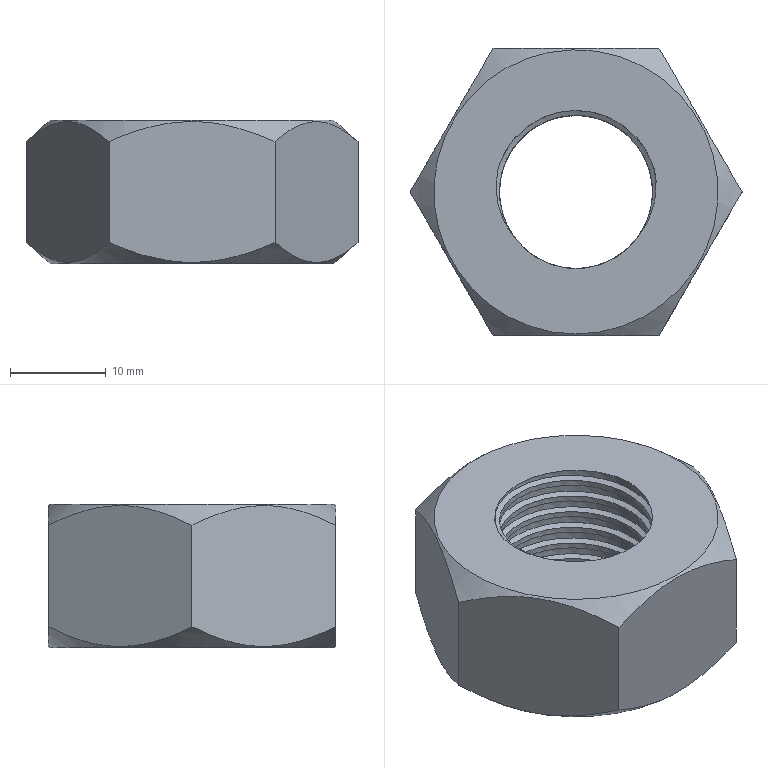Component | NX | 10__NUT_M16X1_5__2_6 | 1 solid | 15 faces | volume 8339 mm3 | plane 9 | cylinder 2 | cone 2 | spline 2 | commonest cylinder face diameters 16 x1 17 x1